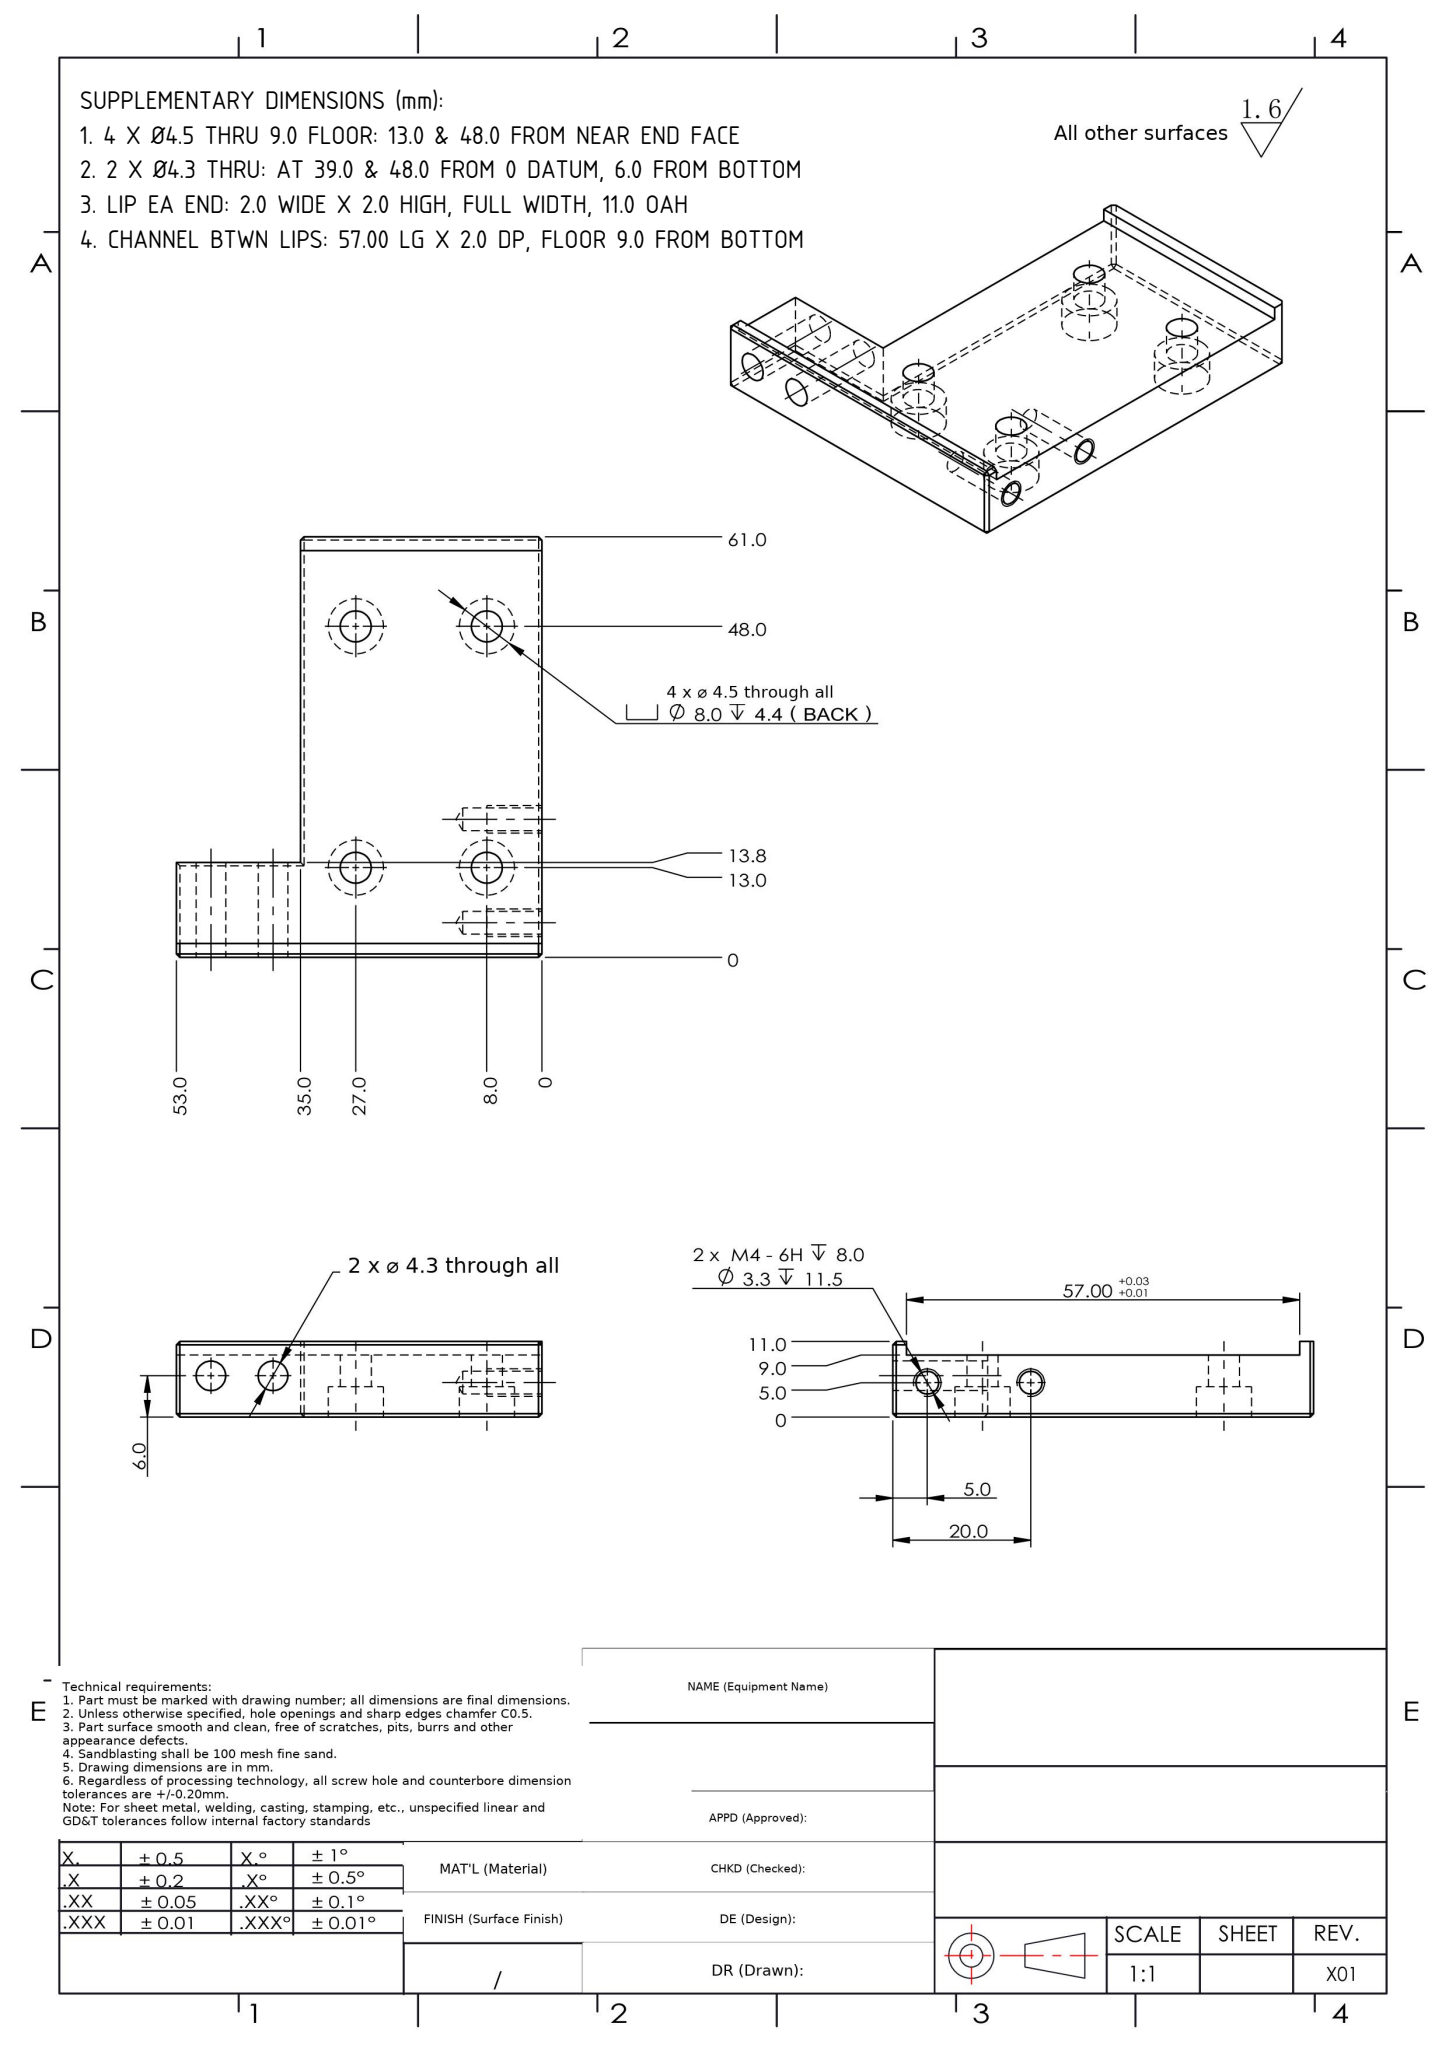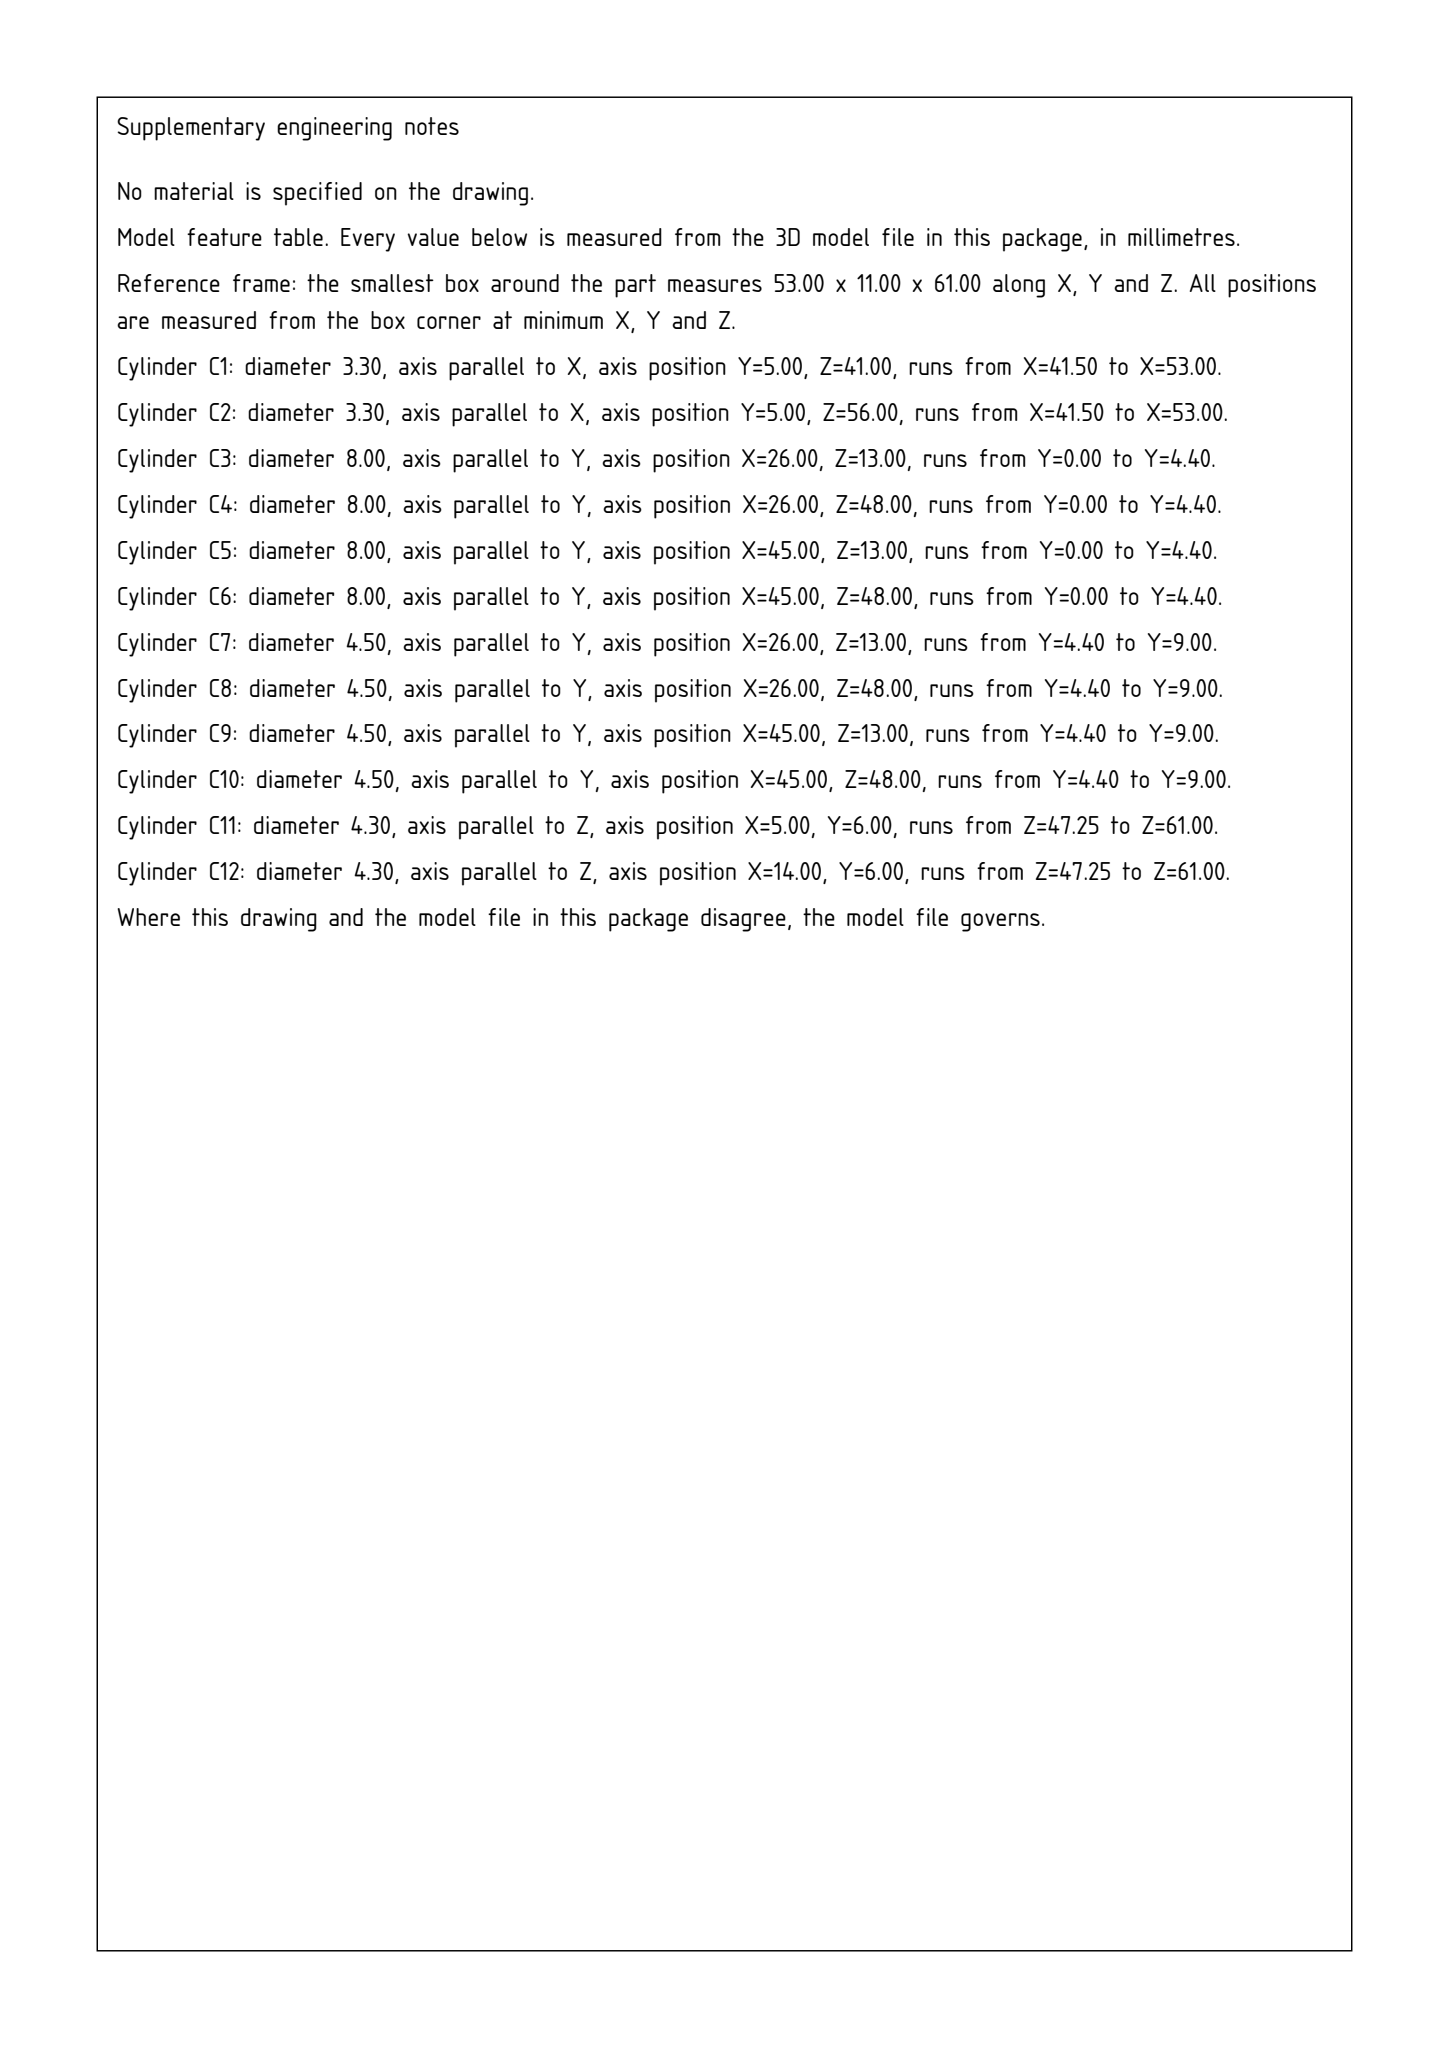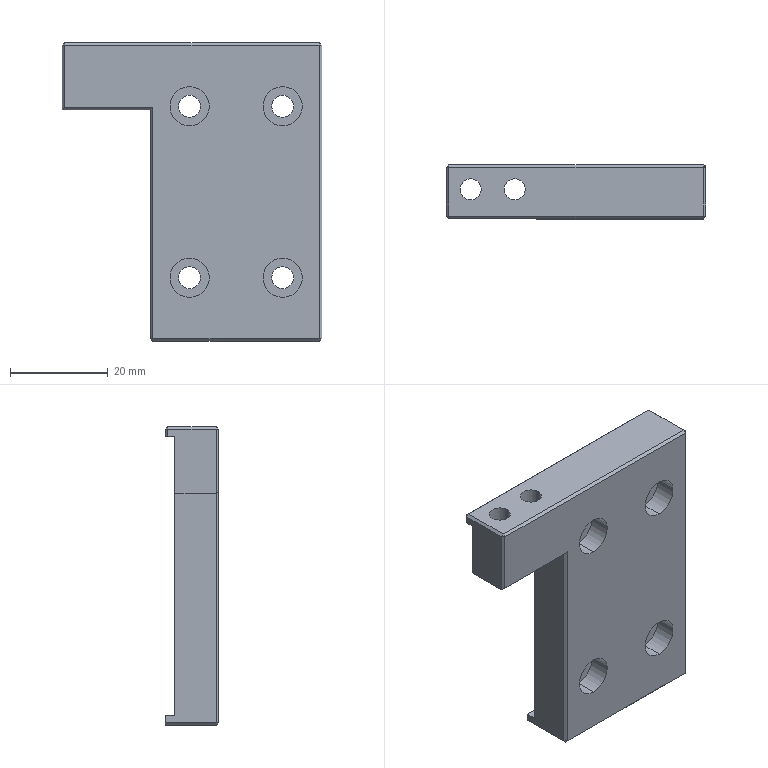Part | SolidWorks | mm | 1 solid | 63 faces | box 53 x 11 x 61 mm | volume 19975 mm3 | plane 35 | cylinder 24 | cone 4 | commonest cylinder face diameters 8 x8 4.5 x8 3.3 x4 4.3 x4
build123d program:
from build123d import *

# Parameters (mm, degrees)
SKETCH3_W                                       = 35
SKETCH3_H                                       = 61
BOSS_EXTRUDE1_DEPTH                             = 11
SKETCH5_W                                       = 35
SKETCH5_H                                       = 57
CUT_EXTRUDE1_DEPTH                              = 2
M4_HEX_SOCKET_HEAD_CAP_SCREW_CBORE1_D           = 4.5
M4_HEX_SOCKET_HEAD_CAP_SCREW_CBORE1_CBORE_D     = 8
M4_HEX_SOCKET_HEAD_CAP_SCREW_CBORE1_CBORE_DEPTH = 4.4
BOSS_EXTRUDE2_DEPTH                             = 18
M4_CLEARANCE_HOLE_1_D                           = 4.3
CHAMFER1_SIZE                                   = 0.5
M4_TAPPED_HOLE1_D                               = 3.3
M4_TAPPED_HOLE1_DEPTH                           = 11.5
M4_TAPPED_HOLE1_TIP                             = 0.9914


with BuildPart() as part:
    # Sketch3 → Boss-Extrude1 (new body)
    with BuildSketch(Plane(origin=(0, 0, 0), x_dir=(1, 0, 0), z_dir=(0, 1, 0))):
        Rectangle(SKETCH3_W, SKETCH3_H)
    extrude(amount=BOSS_EXTRUDE1_DEPTH)

    # Sketch5 → Cut-Extrude1 (cut)
    with BuildSketch(Plane(origin=(0, 11, 0), x_dir=(1, 0, 0), z_dir=(0, 1, 0))):
        Rectangle(SKETCH5_W, SKETCH5_H)
    extrude(amount=-CUT_EXTRUDE1_DEPTH, mode=Mode.SUBTRACT)

    # M4 Hex Socket Head Cap Screw CBORE1 (through all)
    with Locations(Plane(origin=(0, 0, 0), x_dir=(-1, 0, 0), z_dir=(0, -1, 0))):
        with Locations((-9.5, -17.5), (9.5, -17.5), (-9.5, 17.5), (9.5, 17.5)):
            CounterBoreHole(M4_HEX_SOCKET_HEAD_CAP_SCREW_CBORE1_D / 2, M4_HEX_SOCKET_HEAD_CAP_SCREW_CBORE1_CBORE_D / 2, M4_HEX_SOCKET_HEAD_CAP_SCREW_CBORE1_CBORE_DEPTH)

    # Sketch9 → Boss-Extrude2 (add)
    with BuildSketch(Plane.ZY.offset(17.5)):
        Polygon((30.5, 11), (30.5, 0), (16.75, 0), (16.75, 9), (28.5, 9), (28.5, 11), align=None)
    extrude(amount=BOSS_EXTRUDE2_DEPTH)

    # M4 Clearance Hole 1 (through all)
    with Locations(Plane.XY.offset(30.5)):
        with Locations((-21.5, 6), (-30.5, 6)):
            Hole(M4_CLEARANCE_HOLE_1_D / 2)

    # Chamfer1
    chamfer1_edges = [part.edges().sort_by_distance(p)[0] for p in [
        (-9, 11, 30.5),
        (17.5, 11, 29.5),
        (-9, 0, 30.5),
        (-17.5, 0, -6.875),
        (0, 0, -30.5),
        (17.5, 0, 0),
        (-26.5, 0, 16.75),
        (-35.5, 11, 29.5),
        (-35.5, 0, 23.625),
        (-35.5, 5.5, 30.5),
        (17.5, 5.5, 30.5),
        (-17.5, 5.5, -30.5),
        (17.5, 5.5, -30.5),
    ]]
    chamfer(chamfer1_edges, length=CHAMFER1_SIZE)

    # M4 Tapped Hole1
    with Locations(Plane(origin=(17.5, 0, 0), x_dir=(0, 0, -1), z_dir=(1, 0, 0))):
        with Locations((-10.5, 5), (-25.5, 5)):
            Hole(M4_TAPPED_HOLE1_D / 2, depth=M4_TAPPED_HOLE1_DEPTH)
            with Locations((0, 0, -(M4_TAPPED_HOLE1_DEPTH + M4_TAPPED_HOLE1_TIP / 2))):  # 118° drill point
                Cone(0, M4_TAPPED_HOLE1_D / 2, M4_TAPPED_HOLE1_TIP, mode=Mode.SUBTRACT)


solid = part.part